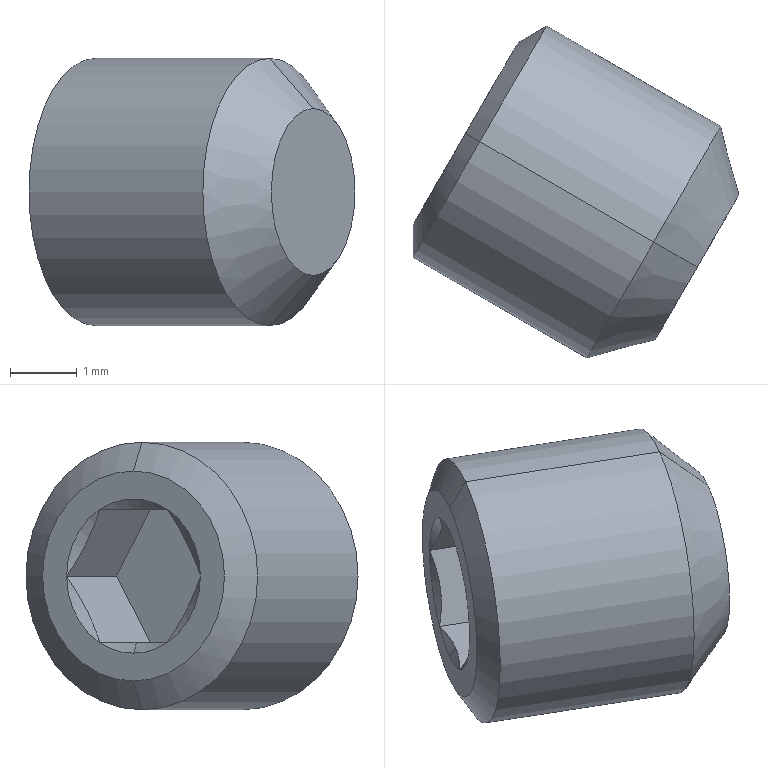Component | SolidWorks | PBT17-2-1_Headless_pin_DIN_913_M4x4-2-2 | 1 solid | 22 faces | box 4.87 x 4.97 x 4 mm | volume 41 mm3 | cone 11 | plane 9 | cylinder 2 | commonest cylinder face diameters 4 x2
STEP:
#1=COLOUR_RGB('',0.7922,0.8196,0.9333);
#2=FILL_AREA_STYLE_COLOUR('',#1);
#3=FILL_AREA_STYLE('',(#2));
#4=SURFACE_STYLE_FILL_AREA(#3);
#5=SURFACE_SIDE_STYLE('',(#4));
#6=SURFACE_STYLE_USAGE(.BOTH.,#5);
#7=PRESENTATION_STYLE_ASSIGNMENT((#6));
#8=CARTESIAN_POINT('',(19.25,-8.991,-6.672));
#9=VERTEX_POINT('',#8);
#10=CARTESIAN_POINT('',(19.25,-8.991,-6.549));
#11=VERTEX_POINT('',#10);
#12=CARTESIAN_POINT('',(19.25,-8.991,-6.61));
#13=DIRECTION('',(-0.866,0.5,-0.));
#14=DIRECTION('',(0.,0.,-1.));
#15=AXIS2_PLACEMENT_3D('',#12,#13,#14);
#16=CIRCLE('',#15,0.06183);
#17=EDGE_CURVE('',#9,#11,#16,.T.);
#18=ORIENTED_EDGE('',*,*,#17,.F.);
#19=CARTESIAN_POINT('',(19.259,-8.996,-6.689));
#20=VERTEX_POINT('',#19);
#21=CARTESIAN_POINT('',(19.25,-8.991,-6.672));
#22=DIRECTION('',(0.433,-0.25,-0.866));
#23=VECTOR('',#22,39.37);
#24=LINE('',#21,#23);
#25=EDGE_CURVE('',#9,#20,#24,.T.);
#26=ORIENTED_EDGE('',*,*,#25,.T.);
#27=CARTESIAN_POINT('',(19.259,-8.996,-6.532));
#28=VERTEX_POINT('',#27);
#29=CARTESIAN_POINT('',(19.259,-8.996,-6.61));
#30=DIRECTION('',(-0.866,0.5,-0.));
#31=DIRECTION('',(0.,0.,-1.));
#32=AXIS2_PLACEMENT_3D('',#29,#30,#31);
#33=CIRCLE('',#32,0.07874);
#34=EDGE_CURVE('',#20,#28,#33,.T.);
#35=ORIENTED_EDGE('',*,*,#34,.T.);
#36=CARTESIAN_POINT('',(19.25,-8.991,-6.549));
#37=DIRECTION('',(0.433,-0.25,0.866));
#38=VECTOR('',#37,39.37);
#39=LINE('',#36,#38);
#40=EDGE_CURVE('',#11,#28,#39,.T.);
#41=ORIENTED_EDGE('',*,*,#40,.F.);
#42=EDGE_LOOP('',(#18,#26,#35,#41));
#43=FACE_OUTER_BOUND('',#42,.T.);
#44=CARTESIAN_POINT('',(19.25,-8.991,-6.61));
#45=DIRECTION('',(0.866,-0.5,0.));
#46=DIRECTION('',(0.,0.,1.));
#47=AXIS2_PLACEMENT_3D('',#44,#45,#46);
#48=CONICAL_SURFACE('',#47,0.06183,1.047);
#49=ADVANCED_FACE('',(#43),#48,.T.);
#50=CARTESIAN_POINT('',(19.361,-9.055,-6.689));
#51=VERTEX_POINT('',#50);
#52=CARTESIAN_POINT('',(19.361,-9.055,-6.532));
#53=VERTEX_POINT('',#52);
#54=CARTESIAN_POINT('',(19.361,-9.055,-6.61));
#55=DIRECTION('',(-0.866,0.5,-0.));
#56=DIRECTION('',(0.,0.,-1.));
#57=AXIS2_PLACEMENT_3D('',#54,#55,#56);
#58=CIRCLE('',#57,0.07874);
#59=EDGE_CURVE('',#51,#53,#58,.T.);
#60=ORIENTED_EDGE('',*,*,#59,.T.);
#61=CARTESIAN_POINT('',(19.273,-9.004,-6.532));
#62=DIRECTION('',(-0.866,0.5,-0.));
#63=VECTOR('',#62,39.37);
#64=LINE('',#61,#63);
#65=EDGE_CURVE('',#53,#28,#64,.T.);
#66=ORIENTED_EDGE('',*,*,#65,.T.);
#67=ORIENTED_EDGE('',*,*,#34,.F.);
#68=CARTESIAN_POINT('',(19.273,-9.004,-6.689));
#69=DIRECTION('',(-0.866,0.5,-0.));
#70=VECTOR('',#69,39.37);
#71=LINE('',#68,#70);
#72=EDGE_CURVE('',#51,#20,#71,.T.);
#73=ORIENTED_EDGE('',*,*,#72,.F.);
#74=EDGE_LOOP('',(#60,#66,#67,#73));
#75=FACE_OUTER_BOUND('',#74,.T.);
#76=CARTESIAN_POINT('',(19.273,-9.004,-6.61));
#77=DIRECTION('',(-0.866,0.5,-0.));
#78=DIRECTION('',(0.,0.,-1.));
#79=AXIS2_PLACEMENT_3D('',#76,#77,#78);
#80=CYLINDRICAL_SURFACE('',#79,0.07874);
#81=ADVANCED_FACE('',(#75),#80,.T.);
#82=CARTESIAN_POINT('',(19.387,-9.069,-6.66));
#83=VERTEX_POINT('',#82);
#84=CARTESIAN_POINT('',(19.387,-9.069,-6.561));
#85=VERTEX_POINT('',#84);
#86=CARTESIAN_POINT('',(19.387,-9.069,-6.61));
#87=DIRECTION('',(-0.866,0.5,-0.));
#88=DIRECTION('',(0.,0.,-1.));
#89=AXIS2_PLACEMENT_3D('',#86,#87,#88);
#90=CIRCLE('',#89,0.04921);
#91=EDGE_CURVE('',#83,#85,#90,.T.);
#92=ORIENTED_EDGE('',*,*,#91,.T.);
#93=CARTESIAN_POINT('',(19.361,-9.055,-6.532));
#94=DIRECTION('',(-0.6124,0.3536,0.7071));
#95=VECTOR('',#94,39.37);
#96=LINE('',#93,#95);
#97=EDGE_CURVE('',#85,#53,#96,.T.);
#98=ORIENTED_EDGE('',*,*,#97,.T.);
#99=ORIENTED_EDGE('',*,*,#59,.F.);
#100=CARTESIAN_POINT('',(19.361,-9.055,-6.689));
#101=DIRECTION('',(-0.6124,0.3536,-0.7071));
#102=VECTOR('',#101,39.37);
#103=LINE('',#100,#102);
#104=EDGE_CURVE('',#83,#51,#103,.T.);
#105=ORIENTED_EDGE('',*,*,#104,.F.);
#106=EDGE_LOOP('',(#92,#98,#99,#105));
#107=FACE_OUTER_BOUND('',#106,.T.);
#108=CARTESIAN_POINT('',(19.361,-9.055,-6.61));
#109=DIRECTION('',(-0.866,0.5,-0.));
#110=DIRECTION('',(0.,0.,-1.));
#111=AXIS2_PLACEMENT_3D('',#108,#109,#110);
#112=CONICAL_SURFACE('',#111,0.07874,0.7854);
#113=ADVANCED_FACE('',(#107),#112,.T.);
#114=CARTESIAN_POINT('',(19.239,-9.01,-6.65));
#115=VERTEX_POINT('',#114);
#116=CARTESIAN_POINT('',(19.253,-8.993,-6.65));
#117=VERTEX_POINT('',#116);
#118=CARTESIAN_POINT('',(19.239,-9.01,-6.65));
#119=CARTESIAN_POINT('',(19.242,-9.008,-6.65));
#120=CARTESIAN_POINT('',(19.244,-9.005,-6.65));
#121=CARTESIAN_POINT('',(19.249,-8.999,-6.65));
#122=CARTESIAN_POINT('',(19.251,-8.996,-6.65));
#123=CARTESIAN_POINT('',(19.253,-8.993,-6.65));
#124=B_SPLINE_CURVE_WITH_KNOTS('',3,(#118,#119,#120,#121,#122,#123),.UNSPECIFIED.,.F.,.F.,(4,2,4),(0.003092,0.003385,0.003677),.UNSPECIFIED.);
#125=EDGE_CURVE('',#115,#117,#124,.T.);
#126=ORIENTED_EDGE('',*,*,#125,.T.);
#127=CARTESIAN_POINT('',(19.25,-8.991,-6.656));
#128=VERTEX_POINT('',#127);
#129=CARTESIAN_POINT('',(19.273,-9.004,-6.61));
#130=DIRECTION('',(-0.433,0.25,-0.866));
#131=VECTOR('',#130,39.37);
#132=LINE('',#129,#131);
#133=EDGE_CURVE('',#117,#128,#132,.T.);
#134=ORIENTED_EDGE('',*,*,#133,.T.);
#135=CARTESIAN_POINT('',(19.25,-8.991,-6.61));
#136=DIRECTION('',(-0.866,0.5,-0.));
#137=DIRECTION('',(0.,0.,-1.));
#138=AXIS2_PLACEMENT_3D('',#135,#136,#137);
#139=CIRCLE('',#138,0.04546);
#140=EDGE_CURVE('',#128,#115,#139,.T.);
#141=ORIENTED_EDGE('',*,*,#140,.T.);
#142=EDGE_LOOP('',(#126,#134,#141));
#143=FACE_OUTER_BOUND('',#142,.T.);
#144=CARTESIAN_POINT('',(-14.822,10.681,-6.61));
#145=DIRECTION('',(-0.866,0.5,-0.));
#146=DIRECTION('',(0.,-0.,-1.));
#147=AXIS2_PLACEMENT_3D('',#144,#145,#146);
#148=CONICAL_SURFACE('',#147,68.191,1.047);
#149=ADVANCED_FACE('',(#143),#148,.F.);
#150=CARTESIAN_POINT('',(19.228,-9.03,-6.61));
#151=VERTEX_POINT('',#150);
#152=CARTESIAN_POINT('',(19.239,-9.01,-6.571));
#153=VERTEX_POINT('',#152);
#154=CARTESIAN_POINT('',(19.25,-8.991,-6.61));
#155=DIRECTION('',(-0.866,0.5,-0.));
#156=DIRECTION('',(0.,0.,-1.));
#157=AXIS2_PLACEMENT_3D('',#154,#155,#156);
#158=CIRCLE('',#157,0.04546);
#159=EDGE_CURVE('',#151,#153,#158,.T.);
#160=ORIENTED_EDGE('',*,*,#159,.T.);
#161=CARTESIAN_POINT('',(19.239,-9.01,-6.571));
#162=CARTESIAN_POINT('',(19.239,-9.015,-6.578));
#163=CARTESIAN_POINT('',(19.238,-9.019,-6.584));
#164=CARTESIAN_POINT('',(19.234,-9.025,-6.597));
#165=CARTESIAN_POINT('',(19.231,-9.028,-6.604));
#166=CARTESIAN_POINT('',(19.228,-9.03,-6.61));
#167=B_SPLINE_CURVE_WITH_KNOTS('',3,(#161,#162,#163,#164,#165,#166),.UNSPECIFIED.,.F.,.F.,(4,2,4),(0.00000024,0.0005833,0.001166),.UNSPECIFIED.);
#168=EDGE_CURVE('',#153,#151,#167,.T.);
#169=ORIENTED_EDGE('',*,*,#168,.T.);
#170=EDGE_LOOP('',(#160,#169));
#171=FACE_OUTER_BOUND('',#170,.T.);
#172=CARTESIAN_POINT('',(-14.822,10.681,-6.61));
#173=DIRECTION('',(-0.866,0.5,-0.));
#174=DIRECTION('',(0.,-0.,-1.));
#175=AXIS2_PLACEMENT_3D('',#172,#173,#174);
#176=CONICAL_SURFACE('',#175,68.191,1.047);
#177=ADVANCED_FACE('',(#171),#176,.F.);
#178=CARTESIAN_POINT('',(19.25,-8.991,-6.61));
#179=DIRECTION('',(-0.866,0.5,-0.));
#180=DIRECTION('',(0.,0.,-1.));
#181=AXIS2_PLACEMENT_3D('',#178,#179,#180);
#182=CIRCLE('',#181,0.04546);
#183=EDGE_CURVE('',#115,#151,#182,.T.);
#184=ORIENTED_EDGE('',*,*,#183,.T.);
#185=CARTESIAN_POINT('',(19.228,-9.03,-6.61));
#186=CARTESIAN_POINT('',(19.231,-9.028,-6.617));
#187=CARTESIAN_POINT('',(19.234,-9.025,-6.623));
#188=CARTESIAN_POINT('',(19.238,-9.019,-6.637));
#189=CARTESIAN_POINT('',(19.239,-9.015,-6.643));
#190=CARTESIAN_POINT('',(19.239,-9.01,-6.65));
#191=B_SPLINE_CURVE_WITH_KNOTS('',3,(#185,#186,#187,#188,#189,#190),.UNSPECIFIED.,.F.,.F.,(4,2,4),(0.00000024,0.0005833,0.001166),.UNSPECIFIED.);
#192=EDGE_CURVE('',#151,#115,#191,.T.);
#193=ORIENTED_EDGE('',*,*,#192,.T.);
#194=EDGE_LOOP('',(#184,#193));
#195=FACE_OUTER_BOUND('',#194,.T.);
#196=CARTESIAN_POINT('',(-14.822,10.681,-6.61));
#197=DIRECTION('',(-0.866,0.5,-0.));
#198=DIRECTION('',(0.,-0.,-1.));
#199=AXIS2_PLACEMENT_3D('',#196,#197,#198);
#200=CONICAL_SURFACE('',#199,68.191,1.047);
#201=ADVANCED_FACE('',(#195),#200,.F.);
#202=ORIENTED_EDGE('',*,*,#133,.F.);
#203=CARTESIAN_POINT('',(19.262,-8.971,-6.65));
#204=VERTEX_POINT('',#203);
#205=CARTESIAN_POINT('',(19.253,-8.993,-6.65));
#206=CARTESIAN_POINT('',(19.257,-8.986,-6.65));
#207=CARTESIAN_POINT('',(19.26,-8.979,-6.65));
#208=CARTESIAN_POINT('',(19.262,-8.971,-6.65));
#209=B_SPLINE_CURVE_WITH_KNOTS('',3,(#205,#206,#207,#208),.UNSPECIFIED.,.F.,.F.,(4,4),(0.003677,0.004261),.UNSPECIFIED.);
#210=EDGE_CURVE('',#117,#204,#209,.T.);
#211=ORIENTED_EDGE('',*,*,#210,.T.);
#212=CARTESIAN_POINT('',(19.25,-8.991,-6.61));
#213=DIRECTION('',(-0.866,0.5,-0.));
#214=DIRECTION('',(0.,0.,-1.));
#215=AXIS2_PLACEMENT_3D('',#212,#213,#214);
#216=CIRCLE('',#215,0.04546);
#217=EDGE_CURVE('',#204,#128,#216,.T.);
#218=ORIENTED_EDGE('',*,*,#217,.T.);
#219=EDGE_LOOP('',(#202,#211,#218));
#220=FACE_OUTER_BOUND('',#219,.T.);
#221=CARTESIAN_POINT('',(-14.822,10.681,-6.61));
#222=DIRECTION('',(-0.866,0.5,-0.));
#223=DIRECTION('',(0.,-0.,-1.));
#224=AXIS2_PLACEMENT_3D('',#221,#222,#223);
#225=CONICAL_SURFACE('',#224,68.191,1.047);
#226=ADVANCED_FACE('',(#220),#225,.F.);
#227=CARTESIAN_POINT('',(19.273,-8.951,-6.61));
#228=VERTEX_POINT('',#227);
#229=CARTESIAN_POINT('',(19.25,-8.991,-6.61));
#230=DIRECTION('',(-0.866,0.5,-0.));
#231=DIRECTION('',(0.,0.,-1.));
#232=AXIS2_PLACEMENT_3D('',#229,#230,#231);
#233=CIRCLE('',#232,0.04546);
#234=EDGE_CURVE('',#228,#204,#233,.T.);
#235=ORIENTED_EDGE('',*,*,#234,.T.);
#236=CARTESIAN_POINT('',(19.262,-8.971,-6.65));
#237=CARTESIAN_POINT('',(19.265,-8.969,-6.643));
#238=CARTESIAN_POINT('',(19.268,-8.966,-6.637));
#239=CARTESIAN_POINT('',(19.272,-8.96,-6.624));
#240=CARTESIAN_POINT('',(19.273,-8.956,-6.617));
#241=CARTESIAN_POINT('',(19.273,-8.951,-6.61));
#242=B_SPLINE_CURVE_WITH_KNOTS('',3,(#236,#237,#238,#239,#240,#241),.UNSPECIFIED.,.F.,.F.,(4,2,4),(0.00000024,0.0005833,0.001166),.UNSPECIFIED.);
#243=EDGE_CURVE('',#204,#228,#242,.T.);
#244=ORIENTED_EDGE('',*,*,#243,.T.);
#245=EDGE_LOOP('',(#235,#244));
#246=FACE_OUTER_BOUND('',#245,.T.);
#247=CARTESIAN_POINT('',(-14.822,10.681,-6.61));
#248=DIRECTION('',(-0.866,0.5,-0.));
#249=DIRECTION('',(0.,-0.,-1.));
#250=AXIS2_PLACEMENT_3D('',#247,#248,#249);
#251=CONICAL_SURFACE('',#250,68.191,1.047);
#252=ADVANCED_FACE('',(#246),#251,.F.);
#253=CARTESIAN_POINT('',(19.262,-8.971,-6.571));
#254=VERTEX_POINT('',#253);
#255=CARTESIAN_POINT('',(19.25,-8.991,-6.61));
#256=DIRECTION('',(-0.866,0.5,-0.));
#257=DIRECTION('',(0.,0.,-1.));
#258=AXIS2_PLACEMENT_3D('',#255,#256,#257);
#259=CIRCLE('',#258,0.04546);
#260=EDGE_CURVE('',#254,#228,#259,.T.);
#261=ORIENTED_EDGE('',*,*,#260,.T.);
#262=CARTESIAN_POINT('',(19.273,-8.951,-6.61));
#263=CARTESIAN_POINT('',(19.273,-8.956,-6.604));
#264=CARTESIAN_POINT('',(19.272,-8.96,-6.598));
#265=CARTESIAN_POINT('',(19.268,-8.966,-6.584));
#266=CARTESIAN_POINT('',(19.265,-8.969,-6.578));
#267=CARTESIAN_POINT('',(19.262,-8.971,-6.571));
#268=B_SPLINE_CURVE_WITH_KNOTS('',3,(#262,#263,#264,#265,#266,#267),.UNSPECIFIED.,.F.,.F.,(4,2,4),(0.00000024,0.0005833,0.001166),.UNSPECIFIED.);
#269=EDGE_CURVE('',#228,#254,#268,.T.);
#270=ORIENTED_EDGE('',*,*,#269,.T.);
#271=EDGE_LOOP('',(#261,#270));
#272=FACE_OUTER_BOUND('',#271,.T.);
#273=CARTESIAN_POINT('',(-14.822,10.681,-6.61));
#274=DIRECTION('',(-0.866,0.5,-0.));
#275=DIRECTION('',(0.,-0.,-1.));
#276=AXIS2_PLACEMENT_3D('',#273,#274,#275);
#277=CONICAL_SURFACE('',#276,68.191,1.047);
#278=ADVANCED_FACE('',(#272),#277,.F.);
#279=CARTESIAN_POINT('',(19.25,-8.991,-6.61));
#280=DIRECTION('',(-0.866,0.5,-0.));
#281=DIRECTION('',(0.,0.,-1.));
#282=AXIS2_PLACEMENT_3D('',#279,#280,#281);
#283=CIRCLE('',#282,0.04546);
#284=EDGE_CURVE('',#153,#254,#283,.T.);
#285=ORIENTED_EDGE('',*,*,#284,.T.);
#286=CARTESIAN_POINT('',(19.262,-8.971,-6.571));
#287=CARTESIAN_POINT('',(19.26,-8.979,-6.571));
#288=CARTESIAN_POINT('',(19.257,-8.986,-6.571));
#289=CARTESIAN_POINT('',(19.251,-8.996,-6.571));
#290=CARTESIAN_POINT('',(19.249,-8.999,-6.571));
#291=CARTESIAN_POINT('',(19.244,-9.005,-6.571));
#292=CARTESIAN_POINT('',(19.242,-9.008,-6.571));
#293=CARTESIAN_POINT('',(19.239,-9.01,-6.571));
#294=B_SPLINE_CURVE_WITH_KNOTS('',3,(#286,#287,#288,#289,#290,#291,#292,#293),.UNSPECIFIED.,.F.,.F.,(4,2,2,4),(0.00099,0.001574,0.001866,0.002158),.UNSPECIFIED.);
#295=EDGE_CURVE('',#254,#153,#294,.T.);
#296=ORIENTED_EDGE('',*,*,#295,.T.);
#297=EDGE_LOOP('',(#285,#296));
#298=FACE_OUTER_BOUND('',#297,.T.);
#299=CARTESIAN_POINT('',(-14.822,10.681,-6.61));
#300=DIRECTION('',(-0.866,0.5,-0.));
#301=DIRECTION('',(0.,-0.,-1.));
#302=AXIS2_PLACEMENT_3D('',#299,#300,#301);
#303=CONICAL_SURFACE('',#302,68.191,1.047);
#304=ADVANCED_FACE('',(#298),#303,.F.);
#305=ORIENTED_EDGE('',*,*,#91,.F.);
#306=CARTESIAN_POINT('',(19.387,-9.069,-6.61));
#307=DIRECTION('',(-0.866,0.5,-0.));
#308=DIRECTION('',(0.,0.,-1.));
#309=AXIS2_PLACEMENT_3D('',#306,#307,#308);
#310=CIRCLE('',#309,0.04921);
#311=EDGE_CURVE('',#85,#83,#310,.T.);
#312=ORIENTED_EDGE('',*,*,#311,.F.);
#313=EDGE_LOOP('',(#305,#312));
#314=FACE_OUTER_BOUND('',#313,.T.);
#315=CARTESIAN_POINT('',(19.387,-9.069,-6.61));
#316=DIRECTION('',(0.866,-0.5,0.));
#317=DIRECTION('',(-0.,0.,1.));
#318=AXIS2_PLACEMENT_3D('',#315,#316,#317);
#319=PLANE('',#318);
#320=ADVANCED_FACE('',(#314),#319,.T.);
#321=ORIENTED_EDGE('',*,*,#97,.F.);
#322=ORIENTED_EDGE('',*,*,#311,.T.);
#323=ORIENTED_EDGE('',*,*,#104,.T.);
#324=CARTESIAN_POINT('',(19.361,-9.055,-6.61));
#325=DIRECTION('',(-0.866,0.5,-0.));
#326=DIRECTION('',(0.,0.,-1.));
#327=AXIS2_PLACEMENT_3D('',#324,#325,#326);
#328=CIRCLE('',#327,0.07874);
#329=EDGE_CURVE('',#53,#51,#328,.T.);
#330=ORIENTED_EDGE('',*,*,#329,.F.);
#331=EDGE_LOOP('',(#321,#322,#323,#330));
#332=FACE_OUTER_BOUND('',#331,.T.);
#333=CARTESIAN_POINT('',(19.361,-9.055,-6.61));
#334=DIRECTION('',(-0.866,0.5,-0.));
#335=DIRECTION('',(0.,0.,-1.));
#336=AXIS2_PLACEMENT_3D('',#333,#334,#335);
#337=CONICAL_SURFACE('',#336,0.07874,0.7854);
#338=ADVANCED_FACE('',(#332),#337,.T.);
#339=ORIENTED_EDGE('',*,*,#65,.F.);
#340=ORIENTED_EDGE('',*,*,#329,.T.);
#341=ORIENTED_EDGE('',*,*,#72,.T.);
#342=CARTESIAN_POINT('',(19.259,-8.996,-6.61));
#343=DIRECTION('',(-0.866,0.5,-0.));
#344=DIRECTION('',(0.,0.,-1.));
#345=AXIS2_PLACEMENT_3D('',#342,#343,#344);
#346=CIRCLE('',#345,0.07874);
#347=EDGE_CURVE('',#28,#20,#346,.T.);
#348=ORIENTED_EDGE('',*,*,#347,.F.);
#349=EDGE_LOOP('',(#339,#340,#341,#348));
#350=FACE_OUTER_BOUND('',#349,.T.);
#351=CARTESIAN_POINT('',(19.273,-9.004,-6.61));
#352=DIRECTION('',(-0.866,0.5,-0.));
#353=DIRECTION('',(0.,0.,-1.));
#354=AXIS2_PLACEMENT_3D('',#351,#352,#353);
#355=CYLINDRICAL_SURFACE('',#354,0.07874);
#356=ADVANCED_FACE('',(#350),#355,.T.);
#357=ORIENTED_EDGE('',*,*,#25,.F.);
#358=CARTESIAN_POINT('',(19.25,-8.991,-6.61));
#359=DIRECTION('',(-0.866,0.5,-0.));
#360=DIRECTION('',(0.,0.,-1.));
#361=AXIS2_PLACEMENT_3D('',#358,#359,#360);
#362=CIRCLE('',#361,0.06183);
#363=EDGE_CURVE('',#11,#9,#362,.T.);
#364=ORIENTED_EDGE('',*,*,#363,.F.);
#365=ORIENTED_EDGE('',*,*,#40,.T.);
#366=ORIENTED_EDGE('',*,*,#347,.T.);
#367=EDGE_LOOP('',(#357,#364,#365,#366));
#368=FACE_OUTER_BOUND('',#367,.T.);
#369=CARTESIAN_POINT('',(19.25,-8.991,-6.61));
#370=DIRECTION('',(0.866,-0.5,0.));
#371=DIRECTION('',(0.,0.,1.));
#372=AXIS2_PLACEMENT_3D('',#369,#370,#371);
#373=CONICAL_SURFACE('',#372,0.06183,1.047);
#374=ADVANCED_FACE('',(#368),#373,.T.);
#375=ORIENTED_EDGE('',*,*,#363,.T.);
#376=ORIENTED_EDGE('',*,*,#17,.T.);
#377=EDGE_LOOP('',(#375,#376));
#378=FACE_OUTER_BOUND('',#377,.T.);
#379=ORIENTED_EDGE('',*,*,#183,.F.);
#380=ORIENTED_EDGE('',*,*,#140,.F.);
#381=ORIENTED_EDGE('',*,*,#217,.F.);
#382=ORIENTED_EDGE('',*,*,#234,.F.);
#383=ORIENTED_EDGE('',*,*,#260,.F.);
#384=ORIENTED_EDGE('',*,*,#284,.F.);
#385=ORIENTED_EDGE('',*,*,#159,.F.);
#386=EDGE_LOOP('',(#379,#380,#381,#382,#383,#384,#385));
#387=FACE_BOUND('',#386,.T.);
#388=CARTESIAN_POINT('',(19.25,-8.991,-6.672));
#389=DIRECTION('',(-0.866,0.5,-0.));
#390=DIRECTION('',(0.,-0.,-1.));
#391=AXIS2_PLACEMENT_3D('',#388,#389,#390);
#392=PLANE('',#391);
#393=ADVANCED_FACE('',(#378,#387),#392,.T.);
#394=CARTESIAN_POINT('',(19.29,-9.04,-6.571));
#395=VERTEX_POINT('',#394);
#396=CARTESIAN_POINT('',(19.29,-9.04,-6.571));
#397=DIRECTION('',(-0.866,0.5,-0.));
#398=VECTOR('',#397,39.37);
#399=LINE('',#396,#398);
#400=EDGE_CURVE('',#395,#153,#399,.T.);
#401=ORIENTED_EDGE('',*,*,#400,.F.);
#402=CARTESIAN_POINT('',(19.279,-9.06,-6.61));
#403=VERTEX_POINT('',#402);
#404=CARTESIAN_POINT('',(19.29,-9.04,-6.571));
#405=DIRECTION('',(-0.25,-0.433,-0.866));
#406=VECTOR('',#405,39.37);
#407=LINE('',#404,#406);
#408=EDGE_CURVE('',#395,#403,#407,.T.);
#409=ORIENTED_EDGE('',*,*,#408,.T.);
#410=CARTESIAN_POINT('',(19.279,-9.06,-6.61));
#411=DIRECTION('',(-0.866,0.5,-0.));
#412=VECTOR('',#411,39.37);
#413=LINE('',#410,#412);
#414=EDGE_CURVE('',#403,#151,#413,.T.);
#415=ORIENTED_EDGE('',*,*,#414,.T.);
#416=ORIENTED_EDGE('',*,*,#168,.F.);
#417=EDGE_LOOP('',(#401,#409,#415,#416));
#418=FACE_OUTER_BOUND('',#417,.T.);
#419=CARTESIAN_POINT('',(19.29,-9.04,-6.571));
#420=DIRECTION('',(0.433,0.75,-0.5));
#421=DIRECTION('',(0.25,0.433,0.866));
#422=AXIS2_PLACEMENT_3D('',#419,#420,#421);
#423=PLANE('',#422);
#424=ADVANCED_FACE('',(#418),#423,.T.);
#425=ORIENTED_EDGE('',*,*,#414,.F.);
#426=CARTESIAN_POINT('',(19.29,-9.04,-6.65));
#427=VERTEX_POINT('',#426);
#428=CARTESIAN_POINT('',(19.279,-9.06,-6.61));
#429=DIRECTION('',(0.25,0.433,-0.866));
#430=VECTOR('',#429,39.37);
#431=LINE('',#428,#430);
#432=EDGE_CURVE('',#403,#427,#431,.T.);
#433=ORIENTED_EDGE('',*,*,#432,.T.);
#434=CARTESIAN_POINT('',(19.29,-9.04,-6.65));
#435=DIRECTION('',(-0.866,0.5,-0.));
#436=VECTOR('',#435,39.37);
#437=LINE('',#434,#436);
#438=EDGE_CURVE('',#427,#115,#437,.T.);
#439=ORIENTED_EDGE('',*,*,#438,.T.);
#440=ORIENTED_EDGE('',*,*,#192,.F.);
#441=EDGE_LOOP('',(#425,#433,#439,#440));
#442=FACE_OUTER_BOUND('',#441,.T.);
#443=CARTESIAN_POINT('',(19.279,-9.06,-6.61));
#444=DIRECTION('',(0.433,0.75,0.5));
#445=DIRECTION('',(-0.25,-0.433,0.866));
#446=AXIS2_PLACEMENT_3D('',#443,#444,#445);
#447=PLANE('',#446);
#448=ADVANCED_FACE('',(#442),#447,.T.);
#449=ORIENTED_EDGE('',*,*,#438,.F.);
#450=CARTESIAN_POINT('',(19.313,-9.001,-6.65));
#451=VERTEX_POINT('',#450);
#452=CARTESIAN_POINT('',(19.29,-9.04,-6.65));
#453=DIRECTION('',(0.5,0.866,0.));
#454=VECTOR('',#453,39.37);
#455=LINE('',#452,#454);
#456=EDGE_CURVE('',#427,#451,#455,.T.);
#457=ORIENTED_EDGE('',*,*,#456,.T.);
#458=CARTESIAN_POINT('',(19.313,-9.001,-6.65));
#459=DIRECTION('',(-0.866,0.5,-0.));
#460=VECTOR('',#459,39.37);
#461=LINE('',#458,#460);
#462=EDGE_CURVE('',#451,#204,#461,.T.);
#463=ORIENTED_EDGE('',*,*,#462,.T.);
#464=ORIENTED_EDGE('',*,*,#210,.F.);
#465=ORIENTED_EDGE('',*,*,#125,.F.);
#466=EDGE_LOOP('',(#449,#457,#463,#464,#465));
#467=FACE_OUTER_BOUND('',#466,.T.);
#468=CARTESIAN_POINT('',(19.29,-9.04,-6.65));
#469=DIRECTION('',(-0.,-0.,1.));
#470=DIRECTION('',(-0.5,-0.866,-0.));
#471=AXIS2_PLACEMENT_3D('',#468,#469,#470);
#472=PLANE('',#471);
#473=ADVANCED_FACE('',(#467),#472,.T.);
#474=ORIENTED_EDGE('',*,*,#462,.F.);
#475=CARTESIAN_POINT('',(19.324,-8.981,-6.61));
#476=VERTEX_POINT('',#475);
#477=CARTESIAN_POINT('',(19.313,-9.001,-6.65));
#478=DIRECTION('',(0.25,0.433,0.866));
#479=VECTOR('',#478,39.37);
#480=LINE('',#477,#479);
#481=EDGE_CURVE('',#451,#476,#480,.T.);
#482=ORIENTED_EDGE('',*,*,#481,.T.);
#483=CARTESIAN_POINT('',(19.324,-8.981,-6.61));
#484=DIRECTION('',(-0.866,0.5,-0.));
#485=VECTOR('',#484,39.37);
#486=LINE('',#483,#485);
#487=EDGE_CURVE('',#476,#228,#486,.T.);
#488=ORIENTED_EDGE('',*,*,#487,.T.);
#489=ORIENTED_EDGE('',*,*,#243,.F.);
#490=EDGE_LOOP('',(#474,#482,#488,#489));
#491=FACE_OUTER_BOUND('',#490,.T.);
#492=CARTESIAN_POINT('',(19.313,-9.001,-6.65));
#493=DIRECTION('',(-0.433,-0.75,0.5));
#494=DIRECTION('',(-0.25,-0.433,-0.866));
#495=AXIS2_PLACEMENT_3D('',#492,#493,#494);
#496=PLANE('',#495);
#497=ADVANCED_FACE('',(#491),#496,.T.);
#498=ORIENTED_EDGE('',*,*,#487,.F.);
#499=CARTESIAN_POINT('',(19.313,-9.001,-6.571));
#500=VERTEX_POINT('',#499);
#501=CARTESIAN_POINT('',(19.324,-8.981,-6.61));
#502=DIRECTION('',(-0.25,-0.433,0.866));
#503=VECTOR('',#502,39.37);
#504=LINE('',#501,#503);
#505=EDGE_CURVE('',#476,#500,#504,.T.);
#506=ORIENTED_EDGE('',*,*,#505,.T.);
#507=CARTESIAN_POINT('',(19.313,-9.001,-6.571));
#508=DIRECTION('',(-0.866,0.5,-0.));
#509=VECTOR('',#508,39.37);
#510=LINE('',#507,#509);
#511=EDGE_CURVE('',#500,#254,#510,.T.);
#512=ORIENTED_EDGE('',*,*,#511,.T.);
#513=ORIENTED_EDGE('',*,*,#269,.F.);
#514=EDGE_LOOP('',(#498,#506,#512,#513));
#515=FACE_OUTER_BOUND('',#514,.T.);
#516=CARTESIAN_POINT('',(19.324,-8.981,-6.61));
#517=DIRECTION('',(-0.433,-0.75,-0.5));
#518=DIRECTION('',(0.25,0.433,-0.866));
#519=AXIS2_PLACEMENT_3D('',#516,#517,#518);
#520=PLANE('',#519);
#521=ADVANCED_FACE('',(#515),#520,.T.);
#522=ORIENTED_EDGE('',*,*,#511,.F.);
#523=CARTESIAN_POINT('',(19.313,-9.001,-6.571));
#524=DIRECTION('',(-0.5,-0.866,-0.));
#525=VECTOR('',#524,39.37);
#526=LINE('',#523,#525);
#527=EDGE_CURVE('',#500,#395,#526,.T.);
#528=ORIENTED_EDGE('',*,*,#527,.T.);
#529=ORIENTED_EDGE('',*,*,#400,.T.);
#530=ORIENTED_EDGE('',*,*,#295,.F.);
#531=EDGE_LOOP('',(#522,#528,#529,#530));
#532=FACE_OUTER_BOUND('',#531,.T.);
#533=CARTESIAN_POINT('',(19.313,-9.001,-6.571));
#534=DIRECTION('',(0.,0.,-1.));
#535=DIRECTION('',(0.5,0.866,0.));
#536=AXIS2_PLACEMENT_3D('',#533,#534,#535);
#537=PLANE('',#536);
#538=ADVANCED_FACE('',(#532),#537,.T.);
#539=ORIENTED_EDGE('',*,*,#408,.F.);
#540=ORIENTED_EDGE('',*,*,#527,.F.);
#541=ORIENTED_EDGE('',*,*,#505,.F.);
#542=ORIENTED_EDGE('',*,*,#481,.F.);
#543=ORIENTED_EDGE('',*,*,#456,.F.);
#544=ORIENTED_EDGE('',*,*,#432,.F.);
#545=EDGE_LOOP('',(#539,#540,#541,#542,#543,#544));
#546=FACE_OUTER_BOUND('',#545,.T.);
#547=CARTESIAN_POINT('',(19.301,-9.02,-6.61));
#548=DIRECTION('',(0.866,-0.5,0.));
#549=DIRECTION('',(0.5,0.866,0.));
#550=AXIS2_PLACEMENT_3D('',#547,#548,#549);
#551=PLANE('',#550);
#552=ADVANCED_FACE('',(#546),#551,.F.);
#553=CLOSED_SHELL('',(#49,#81,#113,#149,#177,#201,#226,#252,#278,#304,#320,#338,#356,#374,#393,#424,#448,#473,#497,#521,#538,#552));
#554=MANIFOLD_SOLID_BREP('',#553);
#555=STYLED_ITEM('',(#7),#554);
#556=PRESENTATION_LAYER_ASSIGNMENT('','',(#555));
#557=CARTESIAN_POINT('',(0.,0.,0.));
#558=DIRECTION('',(0.,0.,1.));
#559=DIRECTION('',(1.,0.,0.));
#560=AXIS2_PLACEMENT_3D('',#557,#558,#559);
#561=(LENGTH_UNIT()NAMED_UNIT(*)SI_UNIT($,.METRE.));
#562=LENGTH_MEASURE_WITH_UNIT(LENGTH_MEASURE(0.0254),#561);
#563=DIMENSIONAL_EXPONENTS(1.,0.,0.,0.,0.,0.,0.);
#564=(CONVERSION_BASED_UNIT('',#562)LENGTH_UNIT()NAMED_UNIT(#563));
#565=UNCERTAINTY_MEASURE_WITH_UNIT(LENGTH_MEASURE(0.00001),#564,'','');
#566=(NAMED_UNIT(*)PLANE_ANGLE_UNIT()SI_UNIT($,.RADIAN.));
#567=(NAMED_UNIT(*)SI_UNIT($,.STERADIAN.)SOLID_ANGLE_UNIT());
#568=(GEOMETRIC_REPRESENTATION_CONTEXT(3)GLOBAL_UNCERTAINTY_ASSIGNED_CONTEXT((#565))GLOBAL_UNIT_ASSIGNED_CONTEXT((#564,#566,#567))REPRESENTATION_CONTEXT('',''));
#569=ADVANCED_BREP_SHAPE_REPRESENTATION('',(#554,#560),#568);
#570=(LENGTH_UNIT()NAMED_UNIT(*)SI_UNIT($,.METRE.));
#571=LENGTH_MEASURE_WITH_UNIT(LENGTH_MEASURE(0.0254),#570);
#572=DIMENSIONAL_EXPONENTS(1.,0.,0.,0.,0.,0.,0.);
#573=(CONVERSION_BASED_UNIT('',#571)LENGTH_UNIT()NAMED_UNIT(#572));
#574=UNCERTAINTY_MEASURE_WITH_UNIT(LENGTH_MEASURE(0.00001),#573,'','');
#575=(NAMED_UNIT(*)PLANE_ANGLE_UNIT()SI_UNIT($,.RADIAN.));
#576=(NAMED_UNIT(*)SI_UNIT($,.STERADIAN.)SOLID_ANGLE_UNIT());
#577=(GEOMETRIC_REPRESENTATION_CONTEXT(3)GLOBAL_UNCERTAINTY_ASSIGNED_CONTEXT((#574))GLOBAL_UNIT_ASSIGNED_CONTEXT((#573,#575,#576))REPRESENTATION_CONTEXT('',''));
#578=MECHANICAL_DESIGN_GEOMETRIC_PRESENTATION_REPRESENTATION('',(#555),#577);